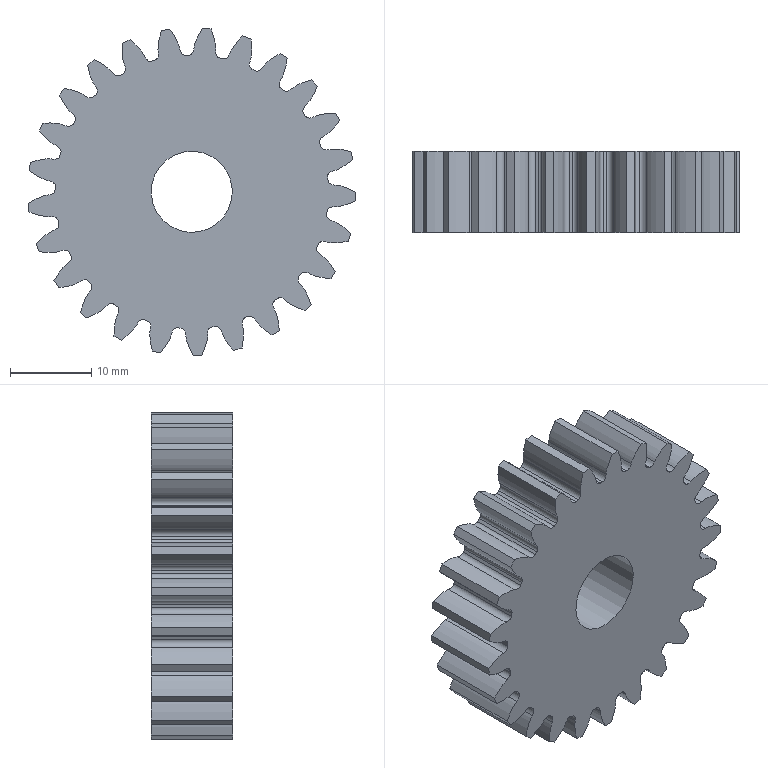Component | NX | JJZ-011 | 1 solid | 153 faces | volume 10066 mm3 | spline 125 | cylinder 26 | plane 2 | commonest cylinder face diameters 33.7 x25 10 x1